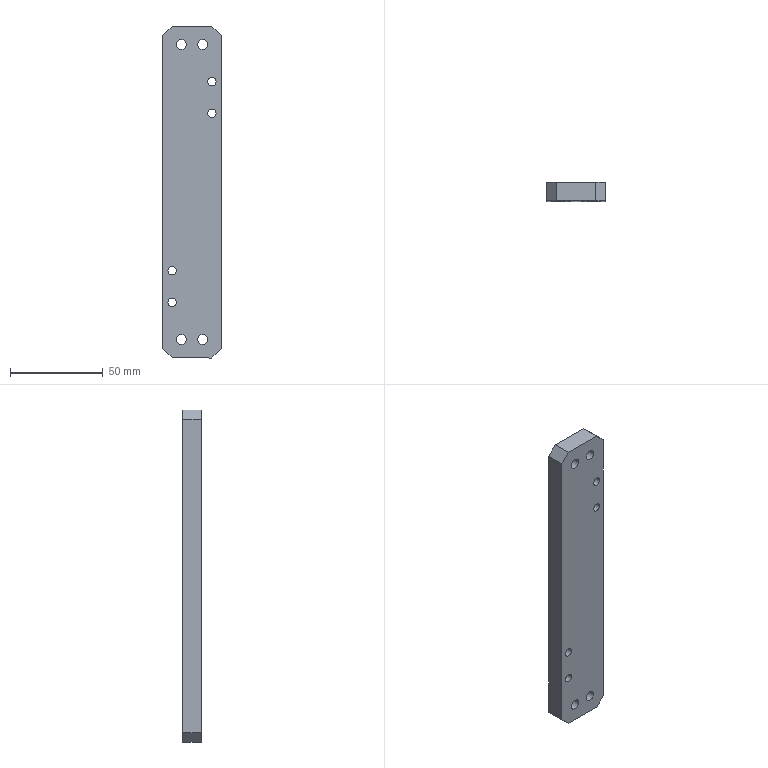Component | SolidWorks | AS-011-JG0129-1 | 1 solid | 26 faces | box 31.5 x 10 x 179 mm | volume 54298 mm3 | cylinder 16 | plane 10 | commonest cylinder face diameters 4.5 x8 5.5 x8
STEP:
#1=COLOUR_RGB('',0.7922,0.8196,0.9333);
#2=FILL_AREA_STYLE_COLOUR('',#1);
#3=FILL_AREA_STYLE('',(#2));
#4=SURFACE_STYLE_FILL_AREA(#3);
#5=SURFACE_SIDE_STYLE('',(#4));
#6=SURFACE_STYLE_USAGE(.BOTH.,#5);
#7=PRESENTATION_STYLE_ASSIGNMENT((#6));
#8=CARTESIAN_POINT('',(-1.289,-3.917,-0.7283));
#9=VERTEX_POINT('',#8);
#10=CARTESIAN_POINT('',(-1.467,-3.917,-0.7283));
#11=VERTEX_POINT('',#10);
#12=CARTESIAN_POINT('',(-1.378,-3.917,-0.7283));
#13=DIRECTION('',(0.,-1.,0.));
#14=DIRECTION('',(1.,0.,0.));
#15=AXIS2_PLACEMENT_3D('',#12,#13,#14);
#16=CIRCLE('',#15,0.08858);
#17=EDGE_CURVE('',#9,#11,#16,.T.);
#18=ORIENTED_EDGE('',*,*,#17,.F.);
#19=CARTESIAN_POINT('',(-1.289,-4.311,-0.7283));
#20=VERTEX_POINT('',#19);
#21=CARTESIAN_POINT('',(-1.289,-3.248,-0.7283));
#22=DIRECTION('',(0.,-1.,0.));
#23=VECTOR('',#22,39.37);
#24=LINE('',#21,#23);
#25=EDGE_CURVE('',#9,#20,#24,.T.);
#26=ORIENTED_EDGE('',*,*,#25,.T.);
#27=CARTESIAN_POINT('',(-1.467,-4.311,-0.7283));
#28=VERTEX_POINT('',#27);
#29=CARTESIAN_POINT('',(-1.378,-4.311,-0.7283));
#30=DIRECTION('',(0.,1.,-0.));
#31=DIRECTION('',(1.,0.,0.));
#32=AXIS2_PLACEMENT_3D('',#29,#30,#31);
#33=CIRCLE('',#32,0.08858);
#34=EDGE_CURVE('',#28,#20,#33,.T.);
#35=ORIENTED_EDGE('',*,*,#34,.F.);
#36=CARTESIAN_POINT('',(-1.467,-3.248,-0.7283));
#37=DIRECTION('',(0.,-1.,0.));
#38=VECTOR('',#37,39.37);
#39=LINE('',#36,#38);
#40=EDGE_CURVE('',#11,#28,#39,.T.);
#41=ORIENTED_EDGE('',*,*,#40,.F.);
#42=EDGE_LOOP('',(#18,#26,#35,#41));
#43=FACE_OUTER_BOUND('',#42,.T.);
#44=CARTESIAN_POINT('',(-1.378,-3.248,-0.7283));
#45=DIRECTION('',(0.,-1.,0.));
#46=DIRECTION('',(-1.,0.,0.));
#47=AXIS2_PLACEMENT_3D('',#44,#45,#46);
#48=CYLINDRICAL_SURFACE('',#47,0.08858);
#49=ADVANCED_FACE('',(#43),#48,.F.);
#50=CARTESIAN_POINT('',(-1.289,-3.917,-0.05906));
#51=VERTEX_POINT('',#50);
#52=CARTESIAN_POINT('',(-1.467,-3.917,-0.05906));
#53=VERTEX_POINT('',#52);
#54=CARTESIAN_POINT('',(-1.378,-3.917,-0.05906));
#55=DIRECTION('',(0.,-1.,0.));
#56=DIRECTION('',(1.,0.,0.));
#57=AXIS2_PLACEMENT_3D('',#54,#55,#56);
#58=CIRCLE('',#57,0.08858);
#59=EDGE_CURVE('',#51,#53,#58,.T.);
#60=ORIENTED_EDGE('',*,*,#59,.F.);
#61=CARTESIAN_POINT('',(-1.289,-4.311,-0.05906));
#62=VERTEX_POINT('',#61);
#63=CARTESIAN_POINT('',(-1.289,-3.248,-0.05906));
#64=DIRECTION('',(0.,-1.,0.));
#65=VECTOR('',#64,39.37);
#66=LINE('',#63,#65);
#67=EDGE_CURVE('',#51,#62,#66,.T.);
#68=ORIENTED_EDGE('',*,*,#67,.T.);
#69=CARTESIAN_POINT('',(-1.467,-4.311,-0.05906));
#70=VERTEX_POINT('',#69);
#71=CARTESIAN_POINT('',(-1.378,-4.311,-0.05906));
#72=DIRECTION('',(0.,1.,-0.));
#73=DIRECTION('',(1.,0.,0.));
#74=AXIS2_PLACEMENT_3D('',#71,#72,#73);
#75=CIRCLE('',#74,0.08858);
#76=EDGE_CURVE('',#70,#62,#75,.T.);
#77=ORIENTED_EDGE('',*,*,#76,.F.);
#78=CARTESIAN_POINT('',(-1.467,-3.248,-0.05906));
#79=DIRECTION('',(0.,-1.,0.));
#80=VECTOR('',#79,39.37);
#81=LINE('',#78,#80);
#82=EDGE_CURVE('',#53,#70,#81,.T.);
#83=ORIENTED_EDGE('',*,*,#82,.F.);
#84=EDGE_LOOP('',(#60,#68,#77,#83));
#85=FACE_OUTER_BOUND('',#84,.T.);
#86=CARTESIAN_POINT('',(-1.378,-3.248,-0.05906));
#87=DIRECTION('',(0.,-1.,0.));
#88=DIRECTION('',(-1.,0.,0.));
#89=AXIS2_PLACEMENT_3D('',#86,#87,#88);
#90=CYLINDRICAL_SURFACE('',#89,0.08858);
#91=ADVANCED_FACE('',(#85),#90,.F.);
#92=CARTESIAN_POINT('',(-2.136,-3.917,-4.075));
#93=VERTEX_POINT('',#92);
#94=CARTESIAN_POINT('',(-2.313,-3.917,-4.075));
#95=VERTEX_POINT('',#94);
#96=CARTESIAN_POINT('',(-2.224,-3.917,-4.075));
#97=DIRECTION('',(0.,-1.,0.));
#98=DIRECTION('',(1.,0.,0.));
#99=AXIS2_PLACEMENT_3D('',#96,#97,#98);
#100=CIRCLE('',#99,0.08858);
#101=EDGE_CURVE('',#93,#95,#100,.T.);
#102=ORIENTED_EDGE('',*,*,#101,.F.);
#103=CARTESIAN_POINT('',(-2.136,-4.311,-4.075));
#104=VERTEX_POINT('',#103);
#105=CARTESIAN_POINT('',(-2.136,-3.248,-4.075));
#106=DIRECTION('',(0.,-1.,0.));
#107=VECTOR('',#106,39.37);
#108=LINE('',#105,#107);
#109=EDGE_CURVE('',#93,#104,#108,.T.);
#110=ORIENTED_EDGE('',*,*,#109,.T.);
#111=CARTESIAN_POINT('',(-2.313,-4.311,-4.075));
#112=VERTEX_POINT('',#111);
#113=CARTESIAN_POINT('',(-2.224,-4.311,-4.075));
#114=DIRECTION('',(0.,1.,-0.));
#115=DIRECTION('',(1.,0.,0.));
#116=AXIS2_PLACEMENT_3D('',#113,#114,#115);
#117=CIRCLE('',#116,0.08858);
#118=EDGE_CURVE('',#112,#104,#117,.T.);
#119=ORIENTED_EDGE('',*,*,#118,.F.);
#120=CARTESIAN_POINT('',(-2.313,-3.248,-4.075));
#121=DIRECTION('',(0.,-1.,0.));
#122=VECTOR('',#121,39.37);
#123=LINE('',#120,#122);
#124=EDGE_CURVE('',#95,#112,#123,.T.);
#125=ORIENTED_EDGE('',*,*,#124,.F.);
#126=EDGE_LOOP('',(#102,#110,#119,#125));
#127=FACE_OUTER_BOUND('',#126,.T.);
#128=CARTESIAN_POINT('',(-2.224,-3.248,-4.075));
#129=DIRECTION('',(0.,-1.,0.));
#130=DIRECTION('',(-1.,0.,0.));
#131=AXIS2_PLACEMENT_3D('',#128,#129,#130);
#132=CYLINDRICAL_SURFACE('',#131,0.08858);
#133=ADVANCED_FACE('',(#127),#132,.F.);
#134=CARTESIAN_POINT('',(-2.136,-3.917,-4.744));
#135=VERTEX_POINT('',#134);
#136=CARTESIAN_POINT('',(-2.313,-3.917,-4.744));
#137=VERTEX_POINT('',#136);
#138=CARTESIAN_POINT('',(-2.224,-3.917,-4.744));
#139=DIRECTION('',(0.,-1.,0.));
#140=DIRECTION('',(1.,0.,0.));
#141=AXIS2_PLACEMENT_3D('',#138,#139,#140);
#142=CIRCLE('',#141,0.08858);
#143=EDGE_CURVE('',#135,#137,#142,.T.);
#144=ORIENTED_EDGE('',*,*,#143,.F.);
#145=CARTESIAN_POINT('',(-2.136,-4.311,-4.744));
#146=VERTEX_POINT('',#145);
#147=CARTESIAN_POINT('',(-2.136,-3.248,-4.744));
#148=DIRECTION('',(0.,-1.,0.));
#149=VECTOR('',#148,39.37);
#150=LINE('',#147,#149);
#151=EDGE_CURVE('',#135,#146,#150,.T.);
#152=ORIENTED_EDGE('',*,*,#151,.T.);
#153=CARTESIAN_POINT('',(-2.313,-4.311,-4.744));
#154=VERTEX_POINT('',#153);
#155=CARTESIAN_POINT('',(-2.224,-4.311,-4.744));
#156=DIRECTION('',(0.,1.,-0.));
#157=DIRECTION('',(1.,0.,0.));
#158=AXIS2_PLACEMENT_3D('',#155,#156,#157);
#159=CIRCLE('',#158,0.08858);
#160=EDGE_CURVE('',#154,#146,#159,.T.);
#161=ORIENTED_EDGE('',*,*,#160,.F.);
#162=CARTESIAN_POINT('',(-2.313,-3.248,-4.744));
#163=DIRECTION('',(0.,-1.,0.));
#164=VECTOR('',#163,39.37);
#165=LINE('',#162,#164);
#166=EDGE_CURVE('',#137,#154,#165,.T.);
#167=ORIENTED_EDGE('',*,*,#166,.F.);
#168=EDGE_LOOP('',(#144,#152,#161,#167));
#169=FACE_OUTER_BOUND('',#168,.T.);
#170=CARTESIAN_POINT('',(-2.224,-3.248,-4.744));
#171=DIRECTION('',(0.,-1.,0.));
#172=DIRECTION('',(-1.,0.,0.));
#173=AXIS2_PLACEMENT_3D('',#170,#171,#172);
#174=CYLINDRICAL_SURFACE('',#173,0.08858);
#175=ADVANCED_FACE('',(#169),#174,.F.);
#176=CARTESIAN_POINT('',(-2.136,-3.917,-5.531));
#177=VERTEX_POINT('',#176);
#178=CARTESIAN_POINT('',(-1.919,-3.917,-5.531));
#179=VERTEX_POINT('',#178);
#180=CARTESIAN_POINT('',(-2.028,-3.917,-5.531));
#181=DIRECTION('',(0.,1.,-0.));
#182=DIRECTION('',(1.,0.,0.));
#183=AXIS2_PLACEMENT_3D('',#180,#181,#182);
#184=CIRCLE('',#183,0.1083);
#185=EDGE_CURVE('',#177,#179,#184,.T.);
#186=ORIENTED_EDGE('',*,*,#185,.T.);
#187=CARTESIAN_POINT('',(-1.919,-4.311,-5.531));
#188=VERTEX_POINT('',#187);
#189=CARTESIAN_POINT('',(-1.919,-3.917,-5.531));
#190=DIRECTION('',(0.,-1.,0.));
#191=VECTOR('',#190,39.37);
#192=LINE('',#189,#191);
#193=EDGE_CURVE('',#179,#188,#192,.T.);
#194=ORIENTED_EDGE('',*,*,#193,.T.);
#195=CARTESIAN_POINT('',(-2.136,-4.311,-5.531));
#196=VERTEX_POINT('',#195);
#197=CARTESIAN_POINT('',(-2.028,-4.311,-5.531));
#198=DIRECTION('',(0.,1.,-0.));
#199=DIRECTION('',(1.,0.,0.));
#200=AXIS2_PLACEMENT_3D('',#197,#198,#199);
#201=CIRCLE('',#200,0.1083);
#202=EDGE_CURVE('',#196,#188,#201,.T.);
#203=ORIENTED_EDGE('',*,*,#202,.F.);
#204=CARTESIAN_POINT('',(-2.136,-3.917,-5.531));
#205=DIRECTION('',(0.,-1.,0.));
#206=VECTOR('',#205,39.37);
#207=LINE('',#204,#206);
#208=EDGE_CURVE('',#177,#196,#207,.T.);
#209=ORIENTED_EDGE('',*,*,#208,.F.);
#210=EDGE_LOOP('',(#186,#194,#203,#209));
#211=FACE_OUTER_BOUND('',#210,.T.);
#212=CARTESIAN_POINT('',(-2.028,-3.917,-5.531));
#213=DIRECTION('',(0.,-1.,0.));
#214=DIRECTION('',(-1.,0.,0.));
#215=AXIS2_PLACEMENT_3D('',#212,#213,#214);
#216=CYLINDRICAL_SURFACE('',#215,0.1083);
#217=ADVANCED_FACE('',(#211),#216,.F.);
#218=CARTESIAN_POINT('',(-1.683,-3.917,-5.531));
#219=VERTEX_POINT('',#218);
#220=CARTESIAN_POINT('',(-1.467,-3.917,-5.531));
#221=VERTEX_POINT('',#220);
#222=CARTESIAN_POINT('',(-1.575,-3.917,-5.531));
#223=DIRECTION('',(0.,1.,-0.));
#224=DIRECTION('',(1.,0.,0.));
#225=AXIS2_PLACEMENT_3D('',#222,#223,#224);
#226=CIRCLE('',#225,0.1083);
#227=EDGE_CURVE('',#219,#221,#226,.T.);
#228=ORIENTED_EDGE('',*,*,#227,.T.);
#229=CARTESIAN_POINT('',(-1.467,-4.311,-5.531));
#230=VERTEX_POINT('',#229);
#231=CARTESIAN_POINT('',(-1.467,-3.917,-5.531));
#232=DIRECTION('',(0.,-1.,0.));
#233=VECTOR('',#232,39.37);
#234=LINE('',#231,#233);
#235=EDGE_CURVE('',#221,#230,#234,.T.);
#236=ORIENTED_EDGE('',*,*,#235,.T.);
#237=CARTESIAN_POINT('',(-1.683,-4.311,-5.531));
#238=VERTEX_POINT('',#237);
#239=CARTESIAN_POINT('',(-1.575,-4.311,-5.531));
#240=DIRECTION('',(0.,1.,-0.));
#241=DIRECTION('',(1.,0.,0.));
#242=AXIS2_PLACEMENT_3D('',#239,#240,#241);
#243=CIRCLE('',#242,0.1083);
#244=EDGE_CURVE('',#238,#230,#243,.T.);
#245=ORIENTED_EDGE('',*,*,#244,.F.);
#246=CARTESIAN_POINT('',(-1.683,-3.917,-5.531));
#247=DIRECTION('',(0.,-1.,0.));
#248=VECTOR('',#247,39.37);
#249=LINE('',#246,#248);
#250=EDGE_CURVE('',#219,#238,#249,.T.);
#251=ORIENTED_EDGE('',*,*,#250,.F.);
#252=EDGE_LOOP('',(#228,#236,#245,#251));
#253=FACE_OUTER_BOUND('',#252,.T.);
#254=CARTESIAN_POINT('',(-1.575,-3.917,-5.531));
#255=DIRECTION('',(0.,-1.,0.));
#256=DIRECTION('',(-1.,0.,0.));
#257=AXIS2_PLACEMENT_3D('',#254,#255,#256);
#258=CYLINDRICAL_SURFACE('',#257,0.1083);
#259=ADVANCED_FACE('',(#253),#258,.F.);
#260=CARTESIAN_POINT('',(-2.136,-3.917,0.7283));
#261=VERTEX_POINT('',#260);
#262=CARTESIAN_POINT('',(-1.919,-3.917,0.7283));
#263=VERTEX_POINT('',#262);
#264=CARTESIAN_POINT('',(-2.028,-3.917,0.7283));
#265=DIRECTION('',(0.,1.,-0.));
#266=DIRECTION('',(1.,0.,0.));
#267=AXIS2_PLACEMENT_3D('',#264,#265,#266);
#268=CIRCLE('',#267,0.1083);
#269=EDGE_CURVE('',#261,#263,#268,.T.);
#270=ORIENTED_EDGE('',*,*,#269,.T.);
#271=CARTESIAN_POINT('',(-1.919,-4.311,0.7283));
#272=VERTEX_POINT('',#271);
#273=CARTESIAN_POINT('',(-1.919,-3.917,0.7283));
#274=DIRECTION('',(0.,-1.,0.));
#275=VECTOR('',#274,39.37);
#276=LINE('',#273,#275);
#277=EDGE_CURVE('',#263,#272,#276,.T.);
#278=ORIENTED_EDGE('',*,*,#277,.T.);
#279=CARTESIAN_POINT('',(-2.136,-4.311,0.7283));
#280=VERTEX_POINT('',#279);
#281=CARTESIAN_POINT('',(-2.028,-4.311,0.7283));
#282=DIRECTION('',(0.,1.,-0.));
#283=DIRECTION('',(1.,0.,0.));
#284=AXIS2_PLACEMENT_3D('',#281,#282,#283);
#285=CIRCLE('',#284,0.1083);
#286=EDGE_CURVE('',#280,#272,#285,.T.);
#287=ORIENTED_EDGE('',*,*,#286,.F.);
#288=CARTESIAN_POINT('',(-2.136,-3.917,0.7283));
#289=DIRECTION('',(0.,-1.,0.));
#290=VECTOR('',#289,39.37);
#291=LINE('',#288,#290);
#292=EDGE_CURVE('',#261,#280,#291,.T.);
#293=ORIENTED_EDGE('',*,*,#292,.F.);
#294=EDGE_LOOP('',(#270,#278,#287,#293));
#295=FACE_OUTER_BOUND('',#294,.T.);
#296=CARTESIAN_POINT('',(-2.028,-3.917,0.7283));
#297=DIRECTION('',(0.,-1.,0.));
#298=DIRECTION('',(-1.,0.,0.));
#299=AXIS2_PLACEMENT_3D('',#296,#297,#298);
#300=CYLINDRICAL_SURFACE('',#299,0.1083);
#301=ADVANCED_FACE('',(#295),#300,.F.);
#302=CARTESIAN_POINT('',(-1.683,-3.917,0.7283));
#303=VERTEX_POINT('',#302);
#304=CARTESIAN_POINT('',(-1.467,-3.917,0.7283));
#305=VERTEX_POINT('',#304);
#306=CARTESIAN_POINT('',(-1.575,-3.917,0.7283));
#307=DIRECTION('',(0.,1.,-0.));
#308=DIRECTION('',(1.,0.,0.));
#309=AXIS2_PLACEMENT_3D('',#306,#307,#308);
#310=CIRCLE('',#309,0.1083);
#311=EDGE_CURVE('',#303,#305,#310,.T.);
#312=ORIENTED_EDGE('',*,*,#311,.T.);
#313=CARTESIAN_POINT('',(-1.467,-4.311,0.7283));
#314=VERTEX_POINT('',#313);
#315=CARTESIAN_POINT('',(-1.467,-3.917,0.7283));
#316=DIRECTION('',(0.,-1.,0.));
#317=VECTOR('',#316,39.37);
#318=LINE('',#315,#317);
#319=EDGE_CURVE('',#305,#314,#318,.T.);
#320=ORIENTED_EDGE('',*,*,#319,.T.);
#321=CARTESIAN_POINT('',(-1.683,-4.311,0.7283));
#322=VERTEX_POINT('',#321);
#323=CARTESIAN_POINT('',(-1.575,-4.311,0.7283));
#324=DIRECTION('',(0.,1.,-0.));
#325=DIRECTION('',(1.,0.,0.));
#326=AXIS2_PLACEMENT_3D('',#323,#324,#325);
#327=CIRCLE('',#326,0.1083);
#328=EDGE_CURVE('',#322,#314,#327,.T.);
#329=ORIENTED_EDGE('',*,*,#328,.F.);
#330=CARTESIAN_POINT('',(-1.683,-3.917,0.7283));
#331=DIRECTION('',(0.,-1.,0.));
#332=VECTOR('',#331,39.37);
#333=LINE('',#330,#332);
#334=EDGE_CURVE('',#303,#322,#333,.T.);
#335=ORIENTED_EDGE('',*,*,#334,.F.);
#336=EDGE_LOOP('',(#312,#320,#329,#335));
#337=FACE_OUTER_BOUND('',#336,.T.);
#338=CARTESIAN_POINT('',(-1.575,-3.917,0.7283));
#339=DIRECTION('',(0.,-1.,0.));
#340=DIRECTION('',(-1.,0.,0.));
#341=AXIS2_PLACEMENT_3D('',#338,#339,#340);
#342=CYLINDRICAL_SURFACE('',#341,0.1083);
#343=ADVANCED_FACE('',(#337),#342,.F.);
#344=ORIENTED_EDGE('',*,*,#76,.T.);
#345=CARTESIAN_POINT('',(-1.378,-4.311,-0.05906));
#346=DIRECTION('',(0.,1.,-0.));
#347=DIRECTION('',(1.,0.,0.));
#348=AXIS2_PLACEMENT_3D('',#345,#346,#347);
#349=CIRCLE('',#348,0.08858);
#350=EDGE_CURVE('',#62,#70,#349,.T.);
#351=ORIENTED_EDGE('',*,*,#350,.T.);
#352=EDGE_LOOP('',(#344,#351));
#353=FACE_BOUND('',#352,.T.);
#354=ORIENTED_EDGE('',*,*,#160,.T.);
#355=CARTESIAN_POINT('',(-2.224,-4.311,-4.744));
#356=DIRECTION('',(0.,1.,-0.));
#357=DIRECTION('',(1.,0.,0.));
#358=AXIS2_PLACEMENT_3D('',#355,#356,#357);
#359=CIRCLE('',#358,0.08858);
#360=EDGE_CURVE('',#146,#154,#359,.T.);
#361=ORIENTED_EDGE('',*,*,#360,.T.);
#362=EDGE_LOOP('',(#354,#361));
#363=FACE_BOUND('',#362,.T.);
#364=CARTESIAN_POINT('',(-1.181,-4.311,-5.728));
#365=VERTEX_POINT('',#364);
#366=CARTESIAN_POINT('',(-1.181,-4.311,0.9252));
#367=VERTEX_POINT('',#366);
#368=CARTESIAN_POINT('',(-1.181,-4.311,-5.925));
#369=DIRECTION('',(0.,0.,1.));
#370=VECTOR('',#369,39.37);
#371=LINE('',#368,#370);
#372=EDGE_CURVE('',#365,#367,#371,.T.);
#373=ORIENTED_EDGE('',*,*,#372,.T.);
#374=CARTESIAN_POINT('',(-1.378,-4.311,1.122));
#375=VERTEX_POINT('',#374);
#376=CARTESIAN_POINT('',(1.934,-4.311,-2.19));
#377=DIRECTION('',(-0.7071,0.,0.7071));
#378=VECTOR('',#377,39.37);
#379=LINE('',#376,#378);
#380=EDGE_CURVE('',#367,#375,#379,.T.);
#381=ORIENTED_EDGE('',*,*,#380,.T.);
#382=CARTESIAN_POINT('',(-2.224,-4.311,1.122));
#383=VERTEX_POINT('',#382);
#384=CARTESIAN_POINT('',(-1.801,-4.311,1.122));
#385=DIRECTION('',(-1.,-0.,-0.));
#386=VECTOR('',#385,39.37);
#387=LINE('',#384,#386);
#388=EDGE_CURVE('',#375,#383,#387,.T.);
#389=ORIENTED_EDGE('',*,*,#388,.T.);
#390=CARTESIAN_POINT('',(-2.421,-4.311,0.9252));
#391=VERTEX_POINT('',#390);
#392=CARTESIAN_POINT('',(-5.536,-4.311,-2.19));
#393=DIRECTION('',(-0.7071,-0.,-0.7071));
#394=VECTOR('',#393,39.37);
#395=LINE('',#392,#394);
#396=EDGE_CURVE('',#383,#391,#395,.T.);
#397=ORIENTED_EDGE('',*,*,#396,.T.);
#398=CARTESIAN_POINT('',(-2.421,-4.311,-5.728));
#399=VERTEX_POINT('',#398);
#400=CARTESIAN_POINT('',(-2.421,-4.311,-5.925));
#401=DIRECTION('',(-0.,-0.,-1.));
#402=VECTOR('',#401,39.37);
#403=LINE('',#400,#402);
#404=EDGE_CURVE('',#391,#399,#403,.T.);
#405=ORIENTED_EDGE('',*,*,#404,.T.);
#406=CARTESIAN_POINT('',(-2.224,-4.311,-5.925));
#407=VERTEX_POINT('',#406);
#408=CARTESIAN_POINT('',(-2.013,-4.311,-6.137));
#409=DIRECTION('',(0.7071,-0.,-0.7071));
#410=VECTOR('',#409,39.37);
#411=LINE('',#408,#410);
#412=EDGE_CURVE('',#399,#407,#411,.T.);
#413=ORIENTED_EDGE('',*,*,#412,.T.);
#414=CARTESIAN_POINT('',(-1.378,-4.311,-5.925));
#415=VERTEX_POINT('',#414);
#416=CARTESIAN_POINT('',(-1.801,-4.311,-5.925));
#417=DIRECTION('',(-1.,0.,0.));
#418=VECTOR('',#417,39.37);
#419=LINE('',#416,#418);
#420=EDGE_CURVE('',#415,#407,#419,.T.);
#421=ORIENTED_EDGE('',*,*,#420,.F.);
#422=CARTESIAN_POINT('',(-1.59,-4.311,-6.137));
#423=DIRECTION('',(0.7071,0.,0.7071));
#424=VECTOR('',#423,39.37);
#425=LINE('',#422,#424);
#426=EDGE_CURVE('',#415,#365,#425,.T.);
#427=ORIENTED_EDGE('',*,*,#426,.T.);
#428=EDGE_LOOP('',(#373,#381,#389,#397,#405,#413,#421,#427));
#429=FACE_OUTER_BOUND('',#428,.T.);
#430=ORIENTED_EDGE('',*,*,#202,.T.);
#431=CARTESIAN_POINT('',(-2.028,-4.311,-5.531));
#432=DIRECTION('',(0.,1.,-0.));
#433=DIRECTION('',(1.,0.,0.));
#434=AXIS2_PLACEMENT_3D('',#431,#432,#433);
#435=CIRCLE('',#434,0.1083);
#436=EDGE_CURVE('',#188,#196,#435,.T.);
#437=ORIENTED_EDGE('',*,*,#436,.T.);
#438=EDGE_LOOP('',(#430,#437));
#439=FACE_BOUND('',#438,.T.);
#440=ORIENTED_EDGE('',*,*,#244,.T.);
#441=CARTESIAN_POINT('',(-1.575,-4.311,-5.531));
#442=DIRECTION('',(0.,1.,-0.));
#443=DIRECTION('',(1.,0.,0.));
#444=AXIS2_PLACEMENT_3D('',#441,#442,#443);
#445=CIRCLE('',#444,0.1083);
#446=EDGE_CURVE('',#230,#238,#445,.T.);
#447=ORIENTED_EDGE('',*,*,#446,.T.);
#448=EDGE_LOOP('',(#440,#447));
#449=FACE_BOUND('',#448,.T.);
#450=ORIENTED_EDGE('',*,*,#286,.T.);
#451=CARTESIAN_POINT('',(-2.028,-4.311,0.7283));
#452=DIRECTION('',(0.,1.,-0.));
#453=DIRECTION('',(1.,0.,0.));
#454=AXIS2_PLACEMENT_3D('',#451,#452,#453);
#455=CIRCLE('',#454,0.1083);
#456=EDGE_CURVE('',#272,#280,#455,.T.);
#457=ORIENTED_EDGE('',*,*,#456,.T.);
#458=EDGE_LOOP('',(#450,#457));
#459=FACE_BOUND('',#458,.T.);
#460=ORIENTED_EDGE('',*,*,#328,.T.);
#461=CARTESIAN_POINT('',(-1.575,-4.311,0.7283));
#462=DIRECTION('',(0.,1.,-0.));
#463=DIRECTION('',(1.,0.,0.));
#464=AXIS2_PLACEMENT_3D('',#461,#462,#463);
#465=CIRCLE('',#464,0.1083);
#466=EDGE_CURVE('',#314,#322,#465,.T.);
#467=ORIENTED_EDGE('',*,*,#466,.T.);
#468=EDGE_LOOP('',(#460,#467));
#469=FACE_BOUND('',#468,.T.);
#470=ORIENTED_EDGE('',*,*,#118,.T.);
#471=CARTESIAN_POINT('',(-2.224,-4.311,-4.075));
#472=DIRECTION('',(0.,1.,-0.));
#473=DIRECTION('',(1.,0.,0.));
#474=AXIS2_PLACEMENT_3D('',#471,#472,#473);
#475=CIRCLE('',#474,0.08858);
#476=EDGE_CURVE('',#104,#112,#475,.T.);
#477=ORIENTED_EDGE('',*,*,#476,.T.);
#478=EDGE_LOOP('',(#470,#477));
#479=FACE_BOUND('',#478,.T.);
#480=ORIENTED_EDGE('',*,*,#34,.T.);
#481=CARTESIAN_POINT('',(-1.378,-4.311,-0.7283));
#482=DIRECTION('',(0.,1.,-0.));
#483=DIRECTION('',(1.,0.,0.));
#484=AXIS2_PLACEMENT_3D('',#481,#482,#483);
#485=CIRCLE('',#484,0.08858);
#486=EDGE_CURVE('',#20,#28,#485,.T.);
#487=ORIENTED_EDGE('',*,*,#486,.T.);
#488=EDGE_LOOP('',(#480,#487));
#489=FACE_BOUND('',#488,.T.);
#490=CARTESIAN_POINT('',(-1.801,-4.311,-5.925));
#491=DIRECTION('',(0.,1.,-0.));
#492=DIRECTION('',(1.,0.,0.));
#493=AXIS2_PLACEMENT_3D('',#490,#491,#492);
#494=PLANE('',#493);
#495=ADVANCED_FACE('',(#353,#363,#429,#439,#449,#459,#469,#479,#489),#494,.F.);
#496=CARTESIAN_POINT('',(-1.378,-3.917,-0.05906));
#497=DIRECTION('',(0.,-1.,0.));
#498=DIRECTION('',(1.,0.,0.));
#499=AXIS2_PLACEMENT_3D('',#496,#497,#498);
#500=CIRCLE('',#499,0.08858);
#501=EDGE_CURVE('',#53,#51,#500,.T.);
#502=ORIENTED_EDGE('',*,*,#501,.T.);
#503=ORIENTED_EDGE('',*,*,#59,.T.);
#504=EDGE_LOOP('',(#502,#503));
#505=FACE_BOUND('',#504,.T.);
#506=CARTESIAN_POINT('',(-2.224,-3.917,-4.744));
#507=DIRECTION('',(0.,-1.,0.));
#508=DIRECTION('',(1.,0.,0.));
#509=AXIS2_PLACEMENT_3D('',#506,#507,#508);
#510=CIRCLE('',#509,0.08858);
#511=EDGE_CURVE('',#137,#135,#510,.T.);
#512=ORIENTED_EDGE('',*,*,#511,.T.);
#513=ORIENTED_EDGE('',*,*,#143,.T.);
#514=EDGE_LOOP('',(#512,#513));
#515=FACE_BOUND('',#514,.T.);
#516=CARTESIAN_POINT('',(-1.181,-3.917,-5.728));
#517=VERTEX_POINT('',#516);
#518=CARTESIAN_POINT('',(-1.181,-3.917,0.9252));
#519=VERTEX_POINT('',#518);
#520=CARTESIAN_POINT('',(-1.181,-3.917,-5.925));
#521=DIRECTION('',(0.,0.,1.));
#522=VECTOR('',#521,39.37);
#523=LINE('',#520,#522);
#524=EDGE_CURVE('',#517,#519,#523,.T.);
#525=ORIENTED_EDGE('',*,*,#524,.F.);
#526=CARTESIAN_POINT('',(-1.378,-3.917,-5.925));
#527=VERTEX_POINT('',#526);
#528=CARTESIAN_POINT('',(-1.59,-3.917,-6.137));
#529=DIRECTION('',(0.7071,0.,0.7071));
#530=VECTOR('',#529,39.37);
#531=LINE('',#528,#530);
#532=EDGE_CURVE('',#527,#517,#531,.T.);
#533=ORIENTED_EDGE('',*,*,#532,.F.);
#534=CARTESIAN_POINT('',(-2.224,-3.917,-5.925));
#535=VERTEX_POINT('',#534);
#536=CARTESIAN_POINT('',(-1.801,-3.917,-5.925));
#537=DIRECTION('',(-1.,0.,0.));
#538=VECTOR('',#537,39.37);
#539=LINE('',#536,#538);
#540=EDGE_CURVE('',#527,#535,#539,.T.);
#541=ORIENTED_EDGE('',*,*,#540,.T.);
#542=CARTESIAN_POINT('',(-2.421,-3.917,-5.728));
#543=VERTEX_POINT('',#542);
#544=CARTESIAN_POINT('',(-2.013,-3.917,-6.137));
#545=DIRECTION('',(0.7071,-0.,-0.7071));
#546=VECTOR('',#545,39.37);
#547=LINE('',#544,#546);
#548=EDGE_CURVE('',#543,#535,#547,.T.);
#549=ORIENTED_EDGE('',*,*,#548,.F.);
#550=CARTESIAN_POINT('',(-2.421,-3.917,0.9252));
#551=VERTEX_POINT('',#550);
#552=CARTESIAN_POINT('',(-2.421,-3.917,-5.925));
#553=DIRECTION('',(-0.,-0.,-1.));
#554=VECTOR('',#553,39.37);
#555=LINE('',#552,#554);
#556=EDGE_CURVE('',#551,#543,#555,.T.);
#557=ORIENTED_EDGE('',*,*,#556,.F.);
#558=CARTESIAN_POINT('',(-2.224,-3.917,1.122));
#559=VERTEX_POINT('',#558);
#560=CARTESIAN_POINT('',(-5.536,-3.917,-2.19));
#561=DIRECTION('',(-0.7071,-0.,-0.7071));
#562=VECTOR('',#561,39.37);
#563=LINE('',#560,#562);
#564=EDGE_CURVE('',#559,#551,#563,.T.);
#565=ORIENTED_EDGE('',*,*,#564,.F.);
#566=CARTESIAN_POINT('',(-1.378,-3.917,1.122));
#567=VERTEX_POINT('',#566);
#568=CARTESIAN_POINT('',(-1.801,-3.917,1.122));
#569=DIRECTION('',(-1.,-0.,-0.));
#570=VECTOR('',#569,39.37);
#571=LINE('',#568,#570);
#572=EDGE_CURVE('',#567,#559,#571,.T.);
#573=ORIENTED_EDGE('',*,*,#572,.F.);
#574=CARTESIAN_POINT('',(1.934,-3.917,-2.19));
#575=DIRECTION('',(-0.7071,0.,0.7071));
#576=VECTOR('',#575,39.37);
#577=LINE('',#574,#576);
#578=EDGE_CURVE('',#519,#567,#577,.T.);
#579=ORIENTED_EDGE('',*,*,#578,.F.);
#580=EDGE_LOOP('',(#525,#533,#541,#549,#557,#565,#573,#579));
#581=FACE_OUTER_BOUND('',#580,.T.);
#582=ORIENTED_EDGE('',*,*,#185,.F.);
#583=CARTESIAN_POINT('',(-2.028,-3.917,-5.531));
#584=DIRECTION('',(0.,1.,-0.));
#585=DIRECTION('',(1.,0.,0.));
#586=AXIS2_PLACEMENT_3D('',#583,#584,#585);
#587=CIRCLE('',#586,0.1083);
#588=EDGE_CURVE('',#179,#177,#587,.T.);
#589=ORIENTED_EDGE('',*,*,#588,.F.);
#590=EDGE_LOOP('',(#582,#589));
#591=FACE_BOUND('',#590,.T.);
#592=ORIENTED_EDGE('',*,*,#227,.F.);
#593=CARTESIAN_POINT('',(-1.575,-3.917,-5.531));
#594=DIRECTION('',(0.,1.,-0.));
#595=DIRECTION('',(1.,0.,0.));
#596=AXIS2_PLACEMENT_3D('',#593,#594,#595);
#597=CIRCLE('',#596,0.1083);
#598=EDGE_CURVE('',#221,#219,#597,.T.);
#599=ORIENTED_EDGE('',*,*,#598,.F.);
#600=EDGE_LOOP('',(#592,#599));
#601=FACE_BOUND('',#600,.T.);
#602=ORIENTED_EDGE('',*,*,#269,.F.);
#603=CARTESIAN_POINT('',(-2.028,-3.917,0.7283));
#604=DIRECTION('',(0.,1.,-0.));
#605=DIRECTION('',(1.,0.,0.));
#606=AXIS2_PLACEMENT_3D('',#603,#604,#605);
#607=CIRCLE('',#606,0.1083);
#608=EDGE_CURVE('',#263,#261,#607,.T.);
#609=ORIENTED_EDGE('',*,*,#608,.F.);
#610=EDGE_LOOP('',(#602,#609));
#611=FACE_BOUND('',#610,.T.);
#612=ORIENTED_EDGE('',*,*,#311,.F.);
#613=CARTESIAN_POINT('',(-1.575,-3.917,0.7283));
#614=DIRECTION('',(0.,1.,-0.));
#615=DIRECTION('',(1.,0.,0.));
#616=AXIS2_PLACEMENT_3D('',#613,#614,#615);
#617=CIRCLE('',#616,0.1083);
#618=EDGE_CURVE('',#305,#303,#617,.T.);
#619=ORIENTED_EDGE('',*,*,#618,.F.);
#620=EDGE_LOOP('',(#612,#619));
#621=FACE_BOUND('',#620,.T.);
#622=CARTESIAN_POINT('',(-2.224,-3.917,-4.075));
#623=DIRECTION('',(0.,-1.,0.));
#624=DIRECTION('',(1.,0.,-0.));
#625=AXIS2_PLACEMENT_3D('',#622,#623,#624);
#626=CIRCLE('',#625,0.08858);
#627=EDGE_CURVE('',#95,#93,#626,.T.);
#628=ORIENTED_EDGE('',*,*,#627,.T.);
#629=ORIENTED_EDGE('',*,*,#101,.T.);
#630=EDGE_LOOP('',(#628,#629));
#631=FACE_BOUND('',#630,.T.);
#632=CARTESIAN_POINT('',(-1.378,-3.917,-0.7283));
#633=DIRECTION('',(0.,-1.,0.));
#634=DIRECTION('',(1.,0.,0.));
#635=AXIS2_PLACEMENT_3D('',#632,#633,#634);
#636=CIRCLE('',#635,0.08858);
#637=EDGE_CURVE('',#11,#9,#636,.T.);
#638=ORIENTED_EDGE('',*,*,#637,.T.);
#639=ORIENTED_EDGE('',*,*,#17,.T.);
#640=EDGE_LOOP('',(#638,#639));
#641=FACE_BOUND('',#640,.T.);
#642=CARTESIAN_POINT('',(-1.801,-3.917,-5.925));
#643=DIRECTION('',(0.,1.,-0.));
#644=DIRECTION('',(1.,0.,0.));
#645=AXIS2_PLACEMENT_3D('',#642,#643,#644);
#646=PLANE('',#645);
#647=ADVANCED_FACE('',(#505,#515,#581,#591,#601,#611,#621,#631,#641),#646,.T.);
#648=ORIENTED_EDGE('',*,*,#404,.F.);
#649=CARTESIAN_POINT('',(-2.421,-3.917,0.9252));
#650=DIRECTION('',(0.,-1.,0.));
#651=VECTOR('',#650,39.37);
#652=LINE('',#649,#651);
#653=EDGE_CURVE('',#551,#391,#652,.T.);
#654=ORIENTED_EDGE('',*,*,#653,.F.);
#655=ORIENTED_EDGE('',*,*,#556,.T.);
#656=CARTESIAN_POINT('',(-2.421,-3.917,-5.728));
#657=DIRECTION('',(0.,-1.,0.));
#658=VECTOR('',#657,39.37);
#659=LINE('',#656,#658);
#660=EDGE_CURVE('',#543,#399,#659,.T.);
#661=ORIENTED_EDGE('',*,*,#660,.T.);
#662=EDGE_LOOP('',(#648,#654,#655,#661));
#663=FACE_OUTER_BOUND('',#662,.T.);
#664=CARTESIAN_POINT('',(-2.421,-3.917,-5.925));
#665=DIRECTION('',(-1.,0.,0.));
#666=DIRECTION('',(0.,1.,-0.));
#667=AXIS2_PLACEMENT_3D('',#664,#665,#666);
#668=PLANE('',#667);
#669=ADVANCED_FACE('',(#663),#668,.T.);
#670=ORIENTED_EDGE('',*,*,#412,.F.);
#671=ORIENTED_EDGE('',*,*,#660,.F.);
#672=ORIENTED_EDGE('',*,*,#548,.T.);
#673=CARTESIAN_POINT('',(-2.224,-3.917,-5.925));
#674=DIRECTION('',(0.,-1.,0.));
#675=VECTOR('',#674,39.37);
#676=LINE('',#673,#675);
#677=EDGE_CURVE('',#535,#407,#676,.T.);
#678=ORIENTED_EDGE('',*,*,#677,.T.);
#679=EDGE_LOOP('',(#670,#671,#672,#678));
#680=FACE_OUTER_BOUND('',#679,.T.);
#681=CARTESIAN_POINT('',(-2.013,-3.917,-6.137));
#682=DIRECTION('',(-0.7071,-0.,-0.7071));
#683=DIRECTION('',(-0.7071,0.,0.7071));
#684=AXIS2_PLACEMENT_3D('',#681,#682,#683);
#685=PLANE('',#684);
#686=ADVANCED_FACE('',(#680),#685,.T.);
#687=ORIENTED_EDGE('',*,*,#420,.T.);
#688=ORIENTED_EDGE('',*,*,#677,.F.);
#689=ORIENTED_EDGE('',*,*,#540,.F.);
#690=CARTESIAN_POINT('',(-1.378,-3.917,-5.925));
#691=DIRECTION('',(0.,-1.,0.));
#692=VECTOR('',#691,39.37);
#693=LINE('',#690,#692);
#694=EDGE_CURVE('',#527,#415,#693,.T.);
#695=ORIENTED_EDGE('',*,*,#694,.T.);
#696=EDGE_LOOP('',(#687,#688,#689,#695));
#697=FACE_OUTER_BOUND('',#696,.T.);
#698=CARTESIAN_POINT('',(-1.801,-3.917,-5.925));
#699=DIRECTION('',(0.,0.,1.));
#700=DIRECTION('',(1.,-0.,-0.));
#701=AXIS2_PLACEMENT_3D('',#698,#699,#700);
#702=PLANE('',#701);
#703=ADVANCED_FACE('',(#697),#702,.F.);
#704=ORIENTED_EDGE('',*,*,#426,.F.);
#705=ORIENTED_EDGE('',*,*,#694,.F.);
#706=ORIENTED_EDGE('',*,*,#532,.T.);
#707=CARTESIAN_POINT('',(-1.181,-3.917,-5.728));
#708=DIRECTION('',(0.,-1.,0.));
#709=VECTOR('',#708,39.37);
#710=LINE('',#707,#709);
#711=EDGE_CURVE('',#517,#365,#710,.T.);
#712=ORIENTED_EDGE('',*,*,#711,.T.);
#713=EDGE_LOOP('',(#704,#705,#706,#712));
#714=FACE_OUTER_BOUND('',#713,.T.);
#715=CARTESIAN_POINT('',(-1.59,-3.917,-6.137));
#716=DIRECTION('',(0.7071,-0.,-0.7071));
#717=DIRECTION('',(-0.7071,-0.,-0.7071));
#718=AXIS2_PLACEMENT_3D('',#715,#716,#717);
#719=PLANE('',#718);
#720=ADVANCED_FACE('',(#714),#719,.T.);
#721=ORIENTED_EDGE('',*,*,#372,.F.);
#722=ORIENTED_EDGE('',*,*,#711,.F.);
#723=ORIENTED_EDGE('',*,*,#524,.T.);
#724=CARTESIAN_POINT('',(-1.181,-3.917,0.9252));
#725=DIRECTION('',(0.,-1.,0.));
#726=VECTOR('',#725,39.37);
#727=LINE('',#724,#726);
#728=EDGE_CURVE('',#519,#367,#727,.T.);
#729=ORIENTED_EDGE('',*,*,#728,.T.);
#730=EDGE_LOOP('',(#721,#722,#723,#729));
#731=FACE_OUTER_BOUND('',#730,.T.);
#732=CARTESIAN_POINT('',(-1.181,-3.917,-5.925));
#733=DIRECTION('',(1.,0.,0.));
#734=DIRECTION('',(0.,-1.,0.));
#735=AXIS2_PLACEMENT_3D('',#732,#733,#734);
#736=PLANE('',#735);
#737=ADVANCED_FACE('',(#731),#736,.T.);
#738=ORIENTED_EDGE('',*,*,#380,.F.);
#739=ORIENTED_EDGE('',*,*,#728,.F.);
#740=ORIENTED_EDGE('',*,*,#578,.T.);
#741=CARTESIAN_POINT('',(-1.378,-3.917,1.122));
#742=DIRECTION('',(0.,-1.,0.));
#743=VECTOR('',#742,39.37);
#744=LINE('',#741,#743);
#745=EDGE_CURVE('',#567,#375,#744,.T.);
#746=ORIENTED_EDGE('',*,*,#745,.T.);
#747=EDGE_LOOP('',(#738,#739,#740,#746));
#748=FACE_OUTER_BOUND('',#747,.T.);
#749=CARTESIAN_POINT('',(1.934,-3.917,-2.19));
#750=DIRECTION('',(0.7071,0.,0.7071));
#751=DIRECTION('',(0.7071,-0.,-0.7071));
#752=AXIS2_PLACEMENT_3D('',#749,#750,#751);
#753=PLANE('',#752);
#754=ADVANCED_FACE('',(#748),#753,.T.);
#755=ORIENTED_EDGE('',*,*,#388,.F.);
#756=ORIENTED_EDGE('',*,*,#745,.F.);
#757=ORIENTED_EDGE('',*,*,#572,.T.);
#758=CARTESIAN_POINT('',(-2.224,-3.917,1.122));
#759=DIRECTION('',(0.,-1.,0.));
#760=VECTOR('',#759,39.37);
#761=LINE('',#758,#760);
#762=EDGE_CURVE('',#559,#383,#761,.T.);
#763=ORIENTED_EDGE('',*,*,#762,.T.);
#764=EDGE_LOOP('',(#755,#756,#757,#763));
#765=FACE_OUTER_BOUND('',#764,.T.);
#766=CARTESIAN_POINT('',(-1.801,-3.917,1.122));
#767=DIRECTION('',(-0.,0.,1.));
#768=DIRECTION('',(1.,0.,0.));
#769=AXIS2_PLACEMENT_3D('',#766,#767,#768);
#770=PLANE('',#769);
#771=ADVANCED_FACE('',(#765),#770,.T.);
#772=ORIENTED_EDGE('',*,*,#396,.F.);
#773=ORIENTED_EDGE('',*,*,#762,.F.);
#774=ORIENTED_EDGE('',*,*,#564,.T.);
#775=ORIENTED_EDGE('',*,*,#653,.T.);
#776=EDGE_LOOP('',(#772,#773,#774,#775));
#777=FACE_OUTER_BOUND('',#776,.T.);
#778=CARTESIAN_POINT('',(-5.536,-3.917,-2.19));
#779=DIRECTION('',(-0.7071,0.,0.7071));
#780=DIRECTION('',(0.7071,0.,0.7071));
#781=AXIS2_PLACEMENT_3D('',#778,#779,#780);
#782=PLANE('',#781);
#783=ADVANCED_FACE('',(#777),#782,.T.);
#784=ORIENTED_EDGE('',*,*,#319,.F.);
#785=ORIENTED_EDGE('',*,*,#618,.T.);
#786=ORIENTED_EDGE('',*,*,#334,.T.);
#787=ORIENTED_EDGE('',*,*,#466,.F.);
#788=EDGE_LOOP('',(#784,#785,#786,#787));
#789=FACE_OUTER_BOUND('',#788,.T.);
#790=CARTESIAN_POINT('',(-1.575,-3.917,0.7283));
#791=DIRECTION('',(0.,-1.,0.));
#792=DIRECTION('',(-1.,0.,0.));
#793=AXIS2_PLACEMENT_3D('',#790,#791,#792);
#794=CYLINDRICAL_SURFACE('',#793,0.1083);
#795=ADVANCED_FACE('',(#789),#794,.F.);
#796=ORIENTED_EDGE('',*,*,#277,.F.);
#797=ORIENTED_EDGE('',*,*,#608,.T.);
#798=ORIENTED_EDGE('',*,*,#292,.T.);
#799=ORIENTED_EDGE('',*,*,#456,.F.);
#800=EDGE_LOOP('',(#796,#797,#798,#799));
#801=FACE_OUTER_BOUND('',#800,.T.);
#802=CARTESIAN_POINT('',(-2.028,-3.917,0.7283));
#803=DIRECTION('',(0.,-1.,0.));
#804=DIRECTION('',(-1.,0.,0.));
#805=AXIS2_PLACEMENT_3D('',#802,#803,#804);
#806=CYLINDRICAL_SURFACE('',#805,0.1083);
#807=ADVANCED_FACE('',(#801),#806,.F.);
#808=ORIENTED_EDGE('',*,*,#235,.F.);
#809=ORIENTED_EDGE('',*,*,#598,.T.);
#810=ORIENTED_EDGE('',*,*,#250,.T.);
#811=ORIENTED_EDGE('',*,*,#446,.F.);
#812=EDGE_LOOP('',(#808,#809,#810,#811));
#813=FACE_OUTER_BOUND('',#812,.T.);
#814=CARTESIAN_POINT('',(-1.575,-3.917,-5.531));
#815=DIRECTION('',(0.,-1.,0.));
#816=DIRECTION('',(-1.,0.,0.));
#817=AXIS2_PLACEMENT_3D('',#814,#815,#816);
#818=CYLINDRICAL_SURFACE('',#817,0.1083);
#819=ADVANCED_FACE('',(#813),#818,.F.);
#820=ORIENTED_EDGE('',*,*,#193,.F.);
#821=ORIENTED_EDGE('',*,*,#588,.T.);
#822=ORIENTED_EDGE('',*,*,#208,.T.);
#823=ORIENTED_EDGE('',*,*,#436,.F.);
#824=EDGE_LOOP('',(#820,#821,#822,#823));
#825=FACE_OUTER_BOUND('',#824,.T.);
#826=CARTESIAN_POINT('',(-2.028,-3.917,-5.531));
#827=DIRECTION('',(0.,-1.,0.));
#828=DIRECTION('',(-1.,0.,0.));
#829=AXIS2_PLACEMENT_3D('',#826,#827,#828);
#830=CYLINDRICAL_SURFACE('',#829,0.1083);
#831=ADVANCED_FACE('',(#825),#830,.F.);
#832=ORIENTED_EDGE('',*,*,#151,.F.);
#833=ORIENTED_EDGE('',*,*,#511,.F.);
#834=ORIENTED_EDGE('',*,*,#166,.T.);
#835=ORIENTED_EDGE('',*,*,#360,.F.);
#836=EDGE_LOOP('',(#832,#833,#834,#835));
#837=FACE_OUTER_BOUND('',#836,.T.);
#838=CARTESIAN_POINT('',(-2.224,-3.248,-4.744));
#839=DIRECTION('',(0.,-1.,0.));
#840=DIRECTION('',(-1.,0.,0.));
#841=AXIS2_PLACEMENT_3D('',#838,#839,#840);
#842=CYLINDRICAL_SURFACE('',#841,0.08858);
#843=ADVANCED_FACE('',(#837),#842,.F.);
#844=ORIENTED_EDGE('',*,*,#109,.F.);
#845=ORIENTED_EDGE('',*,*,#627,.F.);
#846=ORIENTED_EDGE('',*,*,#124,.T.);
#847=ORIENTED_EDGE('',*,*,#476,.F.);
#848=EDGE_LOOP('',(#844,#845,#846,#847));
#849=FACE_OUTER_BOUND('',#848,.T.);
#850=CARTESIAN_POINT('',(-2.224,-3.248,-4.075));
#851=DIRECTION('',(0.,-1.,0.));
#852=DIRECTION('',(-1.,0.,0.));
#853=AXIS2_PLACEMENT_3D('',#850,#851,#852);
#854=CYLINDRICAL_SURFACE('',#853,0.08858);
#855=ADVANCED_FACE('',(#849),#854,.F.);
#856=ORIENTED_EDGE('',*,*,#67,.F.);
#857=ORIENTED_EDGE('',*,*,#501,.F.);
#858=ORIENTED_EDGE('',*,*,#82,.T.);
#859=ORIENTED_EDGE('',*,*,#350,.F.);
#860=EDGE_LOOP('',(#856,#857,#858,#859));
#861=FACE_OUTER_BOUND('',#860,.T.);
#862=CARTESIAN_POINT('',(-1.378,-3.248,-0.05906));
#863=DIRECTION('',(0.,-1.,0.));
#864=DIRECTION('',(-1.,0.,0.));
#865=AXIS2_PLACEMENT_3D('',#862,#863,#864);
#866=CYLINDRICAL_SURFACE('',#865,0.08858);
#867=ADVANCED_FACE('',(#861),#866,.F.);
#868=ORIENTED_EDGE('',*,*,#25,.F.);
#869=ORIENTED_EDGE('',*,*,#637,.F.);
#870=ORIENTED_EDGE('',*,*,#40,.T.);
#871=ORIENTED_EDGE('',*,*,#486,.F.);
#872=EDGE_LOOP('',(#868,#869,#870,#871));
#873=FACE_OUTER_BOUND('',#872,.T.);
#874=CARTESIAN_POINT('',(-1.378,-3.248,-0.7283));
#875=DIRECTION('',(0.,-1.,0.));
#876=DIRECTION('',(-1.,0.,0.));
#877=AXIS2_PLACEMENT_3D('',#874,#875,#876);
#878=CYLINDRICAL_SURFACE('',#877,0.08858);
#879=ADVANCED_FACE('',(#873),#878,.F.);
#880=CLOSED_SHELL('',(#49,#91,#133,#175,#217,#259,#301,#343,#495,#647,#669,#686,#703,#720,#737,#754,#771,#783,#795,#807,#819,#831,#843,#855,#867,#879));
#881=MANIFOLD_SOLID_BREP('',#880);
#882=STYLED_ITEM('',(#7),#881);
#883=(LENGTH_UNIT()NAMED_UNIT(*)SI_UNIT($,.METRE.));
#884=LENGTH_MEASURE_WITH_UNIT(LENGTH_MEASURE(0.0254),#883);
#885=DIMENSIONAL_EXPONENTS(1.,0.,0.,0.,0.,0.,0.);
#886=(CONVERSION_BASED_UNIT('',#884)LENGTH_UNIT()NAMED_UNIT(#885));
#887=UNCERTAINTY_MEASURE_WITH_UNIT(LENGTH_MEASURE(0.00001),#886,'','');
#888=(NAMED_UNIT(*)PLANE_ANGLE_UNIT()SI_UNIT($,.RADIAN.));
#889=(NAMED_UNIT(*)SI_UNIT($,.STERADIAN.)SOLID_ANGLE_UNIT());
#890=(GEOMETRIC_REPRESENTATION_CONTEXT(3)GLOBAL_UNCERTAINTY_ASSIGNED_CONTEXT((#887))GLOBAL_UNIT_ASSIGNED_CONTEXT((#886,#888,#889))REPRESENTATION_CONTEXT('',''));
#891=MECHANICAL_DESIGN_GEOMETRIC_PRESENTATION_REPRESENTATION('',(#882),#890);
#892=PRESENTATION_LAYER_ASSIGNMENT('','',(#882));
#893=CARTESIAN_POINT('',(0.,0.,0.));
#894=DIRECTION('',(0.,0.,1.));
#895=DIRECTION('',(1.,0.,0.));
#896=AXIS2_PLACEMENT_3D('',#893,#894,#895);
#897=(LENGTH_UNIT()NAMED_UNIT(*)SI_UNIT($,.METRE.));
#898=LENGTH_MEASURE_WITH_UNIT(LENGTH_MEASURE(0.0254),#897);
#899=DIMENSIONAL_EXPONENTS(1.,0.,0.,0.,0.,0.,0.);
#900=(CONVERSION_BASED_UNIT('',#898)LENGTH_UNIT()NAMED_UNIT(#899));
#901=UNCERTAINTY_MEASURE_WITH_UNIT(LENGTH_MEASURE(0.00001),#900,'','');
#902=(NAMED_UNIT(*)PLANE_ANGLE_UNIT()SI_UNIT($,.RADIAN.));
#903=(NAMED_UNIT(*)SI_UNIT($,.STERADIAN.)SOLID_ANGLE_UNIT());
#904=(GEOMETRIC_REPRESENTATION_CONTEXT(3)GLOBAL_UNCERTAINTY_ASSIGNED_CONTEXT((#901))GLOBAL_UNIT_ASSIGNED_CONTEXT((#900,#902,#903))REPRESENTATION_CONTEXT('',''));
#905=ADVANCED_BREP_SHAPE_REPRESENTATION('',(#881,#896),#904);